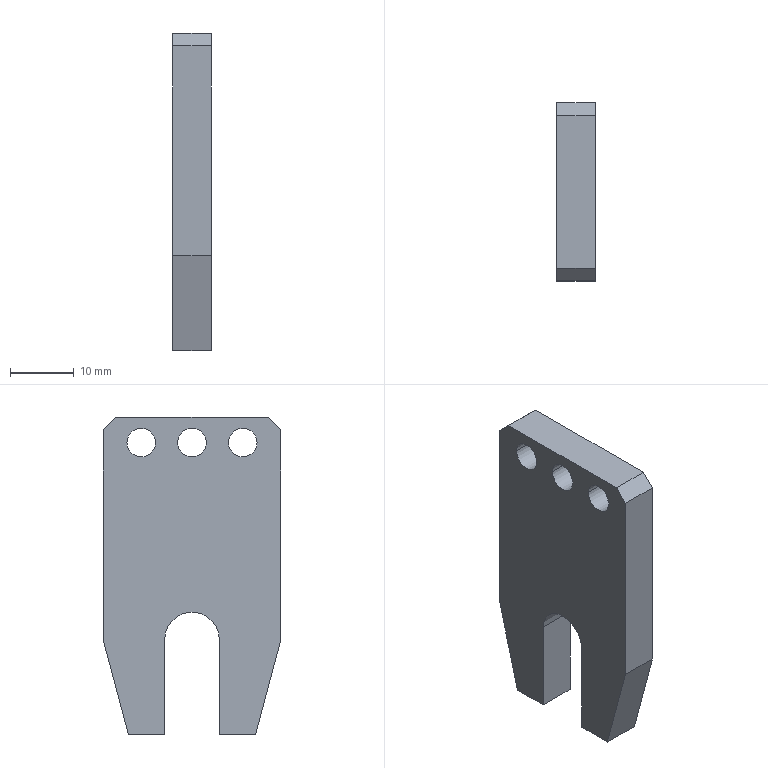Component | SolidWorks | 09HHHHHH4-1 | 1 solid | 20 faces | box 6 x 28 x 50 mm | volume 6781 mm3 | plane 13 | cylinder 7 | commonest cylinder face diameters 4.5 x6 8.6 x1
build123d program:
from build123d import *

# Parameters (mm, degrees)
SKETCH1_W           = 28
SKETCH1_H           = 50
BOSS_EXTRUDE1_DEPTH = 6
CUT_EXTRUDE1_DEPTH  = 324.627
CHAMFER1_SIZE       = 2
SKETCH3_R           = 2.25
CUT_EXTRUDE2_DEPTH  = 324.627


with BuildPart() as part:
    # Sketch1 → Boss-Extrude1 (new body)
    with BuildSketch(Plane.XY):
        with Locations((306.066, -22.5)):
            Rectangle(SKETCH1_W, SKETCH1_H)
    extrude(amount=BOSS_EXTRUDE1_DEPTH)

    # Sketch2 → Cut-Extrude1 (cut, through all)
    with BuildSketch(Plane.XY.offset(6)):
        with BuildLine():
            Line((310.366, -32.5), (310.366, -47.5))
            ThreePointArc((310.366, -47.5), (306.066, -51.8), (301.766, -47.5))
            Line((301.766, -47.5), (301.766, -32.5))
            ThreePointArc((301.766, -32.5), (306.066, -28.2), (310.366, -32.5))
        make_face()
        Polygon((296.066, -47.5), (292.066, -32.5), (292.066, -47.5), align=None)
        Polygon((320.066, -47.5), (316.066, -47.5), (320.066, -32.5), align=None)
    extrude(amount=-CUT_EXTRUDE1_DEPTH, mode=Mode.SUBTRACT)

    # Chamfer1
    chamfer1_edges = [part.edges().sort_by_distance(p)[0] for p in [
        (292.066, 2.5, 3),
        (320.066, 2.5, 3),
    ]]
    chamfer(chamfer1_edges, length=CHAMFER1_SIZE)

    # Sketch3 → Cut-Extrude2 (cut, through all)
    with BuildSketch(Plane.XY.offset(6)):
        with Locations((298.066, -1.5)):
            Circle(SKETCH3_R)
        with Locations(Location((314.066, -1.5, 0), (0, 0, 180))):
            Circle(SKETCH3_R)
        with Locations((306.066, -1.5)):
            Circle(SKETCH3_R)
    extrude(amount=-CUT_EXTRUDE2_DEPTH, mode=Mode.SUBTRACT)


solid = part.part

# Placed as in the assembly
solid = solid.moved(Location((-650.94, 19.683, 6.344), (90, -90, 0)))
STEP:
#1=CARTESIAN_POINT('',(-25.628,-11.186,0.1907));
#2=VERTEX_POINT('',#1);
#3=CARTESIAN_POINT('',(-25.628,-11.364,0.1907));
#4=VERTEX_POINT('',#3);
#5=CARTESIAN_POINT('',(-25.628,-11.275,0.1907));
#6=DIRECTION('',(-1.,0.,0.));
#7=DIRECTION('',(0.,-1.,0.));
#8=AXIS2_PLACEMENT_3D('',#5,#6,#7);
#9=CIRCLE('',#8,0.08858);
#10=EDGE_CURVE('',#2,#4,#9,.T.);
#11=ORIENTED_EDGE('',*,*,#10,.F.);
#12=CARTESIAN_POINT('',(-25.864,-11.186,0.1907));
#13=VERTEX_POINT('',#12);
#14=CARTESIAN_POINT('',(-25.628,-11.186,0.1907));
#15=DIRECTION('',(-1.,0.,0.));
#16=VECTOR('',#15,39.37);
#17=LINE('',#14,#16);
#18=EDGE_CURVE('',#2,#13,#17,.T.);
#19=ORIENTED_EDGE('',*,*,#18,.T.);
#20=CARTESIAN_POINT('',(-25.864,-11.364,0.1907));
#21=VERTEX_POINT('',#20);
#22=CARTESIAN_POINT('',(-25.864,-11.275,0.1907));
#23=DIRECTION('',(-1.,0.,0.));
#24=DIRECTION('',(0.,-1.,0.));
#25=AXIS2_PLACEMENT_3D('',#22,#23,#24);
#26=CIRCLE('',#25,0.08858);
#27=EDGE_CURVE('',#13,#21,#26,.T.);
#28=ORIENTED_EDGE('',*,*,#27,.T.);
#29=CARTESIAN_POINT('',(-25.628,-11.364,0.1907));
#30=DIRECTION('',(-1.,0.,0.));
#31=VECTOR('',#30,39.37);
#32=LINE('',#29,#31);
#33=EDGE_CURVE('',#4,#21,#32,.T.);
#34=ORIENTED_EDGE('',*,*,#33,.F.);
#35=EDGE_LOOP('',(#11,#19,#28,#34));
#36=FACE_OUTER_BOUND('',#35,.T.);
#37=CARTESIAN_POINT('',(-25.628,-11.275,0.1907));
#38=DIRECTION('',(-1.,0.,0.));
#39=DIRECTION('',(0.,-1.,0.));
#40=AXIS2_PLACEMENT_3D('',#37,#38,#39);
#41=CYLINDRICAL_SURFACE('',#40,0.08858);
#42=ADVANCED_FACE('',(#36),#41,.F.);
#43=CARTESIAN_POINT('',(-25.628,-11.501,0.1907));
#44=VERTEX_POINT('',#43);
#45=CARTESIAN_POINT('',(-25.628,-11.678,0.1907));
#46=VERTEX_POINT('',#45);
#47=CARTESIAN_POINT('',(-25.628,-11.59,0.1907));
#48=DIRECTION('',(-1.,0.,0.));
#49=DIRECTION('',(0.,1.,0.));
#50=AXIS2_PLACEMENT_3D('',#47,#48,#49);
#51=CIRCLE('',#50,0.08858);
#52=EDGE_CURVE('',#44,#46,#51,.T.);
#53=ORIENTED_EDGE('',*,*,#52,.F.);
#54=CARTESIAN_POINT('',(-25.864,-11.501,0.1907));
#55=VERTEX_POINT('',#54);
#56=CARTESIAN_POINT('',(-25.628,-11.501,0.1907));
#57=DIRECTION('',(-1.,0.,0.));
#58=VECTOR('',#57,39.37);
#59=LINE('',#56,#58);
#60=EDGE_CURVE('',#44,#55,#59,.T.);
#61=ORIENTED_EDGE('',*,*,#60,.T.);
#62=CARTESIAN_POINT('',(-25.864,-11.678,0.1907));
#63=VERTEX_POINT('',#62);
#64=CARTESIAN_POINT('',(-25.864,-11.59,0.1907));
#65=DIRECTION('',(-1.,0.,0.));
#66=DIRECTION('',(0.,1.,0.));
#67=AXIS2_PLACEMENT_3D('',#64,#65,#66);
#68=CIRCLE('',#67,0.08858);
#69=EDGE_CURVE('',#55,#63,#68,.T.);
#70=ORIENTED_EDGE('',*,*,#69,.T.);
#71=CARTESIAN_POINT('',(-25.628,-11.678,0.1907));
#72=DIRECTION('',(-1.,0.,0.));
#73=VECTOR('',#72,39.37);
#74=LINE('',#71,#73);
#75=EDGE_CURVE('',#46,#63,#74,.T.);
#76=ORIENTED_EDGE('',*,*,#75,.F.);
#77=EDGE_LOOP('',(#53,#61,#70,#76));
#78=FACE_OUTER_BOUND('',#77,.T.);
#79=CARTESIAN_POINT('',(-25.628,-11.59,0.1907));
#80=DIRECTION('',(-1.,0.,0.));
#81=DIRECTION('',(0.,-1.,0.));
#82=AXIS2_PLACEMENT_3D('',#79,#80,#81);
#83=CYLINDRICAL_SURFACE('',#82,0.08858);
#84=ADVANCED_FACE('',(#78),#83,.F.);
#85=CARTESIAN_POINT('',(-25.628,-10.871,0.1907));
#86=VERTEX_POINT('',#85);
#87=CARTESIAN_POINT('',(-25.628,-11.049,0.1907));
#88=VERTEX_POINT('',#87);
#89=CARTESIAN_POINT('',(-25.628,-10.96,0.1907));
#90=DIRECTION('',(-1.,0.,0.));
#91=DIRECTION('',(0.,-1.,0.));
#92=AXIS2_PLACEMENT_3D('',#89,#90,#91);
#93=CIRCLE('',#92,0.08858);
#94=EDGE_CURVE('',#86,#88,#93,.T.);
#95=ORIENTED_EDGE('',*,*,#94,.F.);
#96=CARTESIAN_POINT('',(-25.864,-10.871,0.1907));
#97=VERTEX_POINT('',#96);
#98=CARTESIAN_POINT('',(-25.628,-10.871,0.1907));
#99=DIRECTION('',(-1.,0.,0.));
#100=VECTOR('',#99,39.37);
#101=LINE('',#98,#100);
#102=EDGE_CURVE('',#86,#97,#101,.T.);
#103=ORIENTED_EDGE('',*,*,#102,.T.);
#104=CARTESIAN_POINT('',(-25.864,-11.049,0.1907));
#105=VERTEX_POINT('',#104);
#106=CARTESIAN_POINT('',(-25.864,-10.96,0.1907));
#107=DIRECTION('',(-1.,0.,0.));
#108=DIRECTION('',(0.,-1.,0.));
#109=AXIS2_PLACEMENT_3D('',#106,#107,#108);
#110=CIRCLE('',#109,0.08858);
#111=EDGE_CURVE('',#97,#105,#110,.T.);
#112=ORIENTED_EDGE('',*,*,#111,.T.);
#113=CARTESIAN_POINT('',(-25.628,-11.049,0.1907));
#114=DIRECTION('',(-1.,0.,0.));
#115=VECTOR('',#114,39.37);
#116=LINE('',#113,#115);
#117=EDGE_CURVE('',#88,#105,#116,.T.);
#118=ORIENTED_EDGE('',*,*,#117,.F.);
#119=EDGE_LOOP('',(#95,#103,#112,#118));
#120=FACE_OUTER_BOUND('',#119,.T.);
#121=CARTESIAN_POINT('',(-25.628,-10.96,0.1907));
#122=DIRECTION('',(-1.,0.,0.));
#123=DIRECTION('',(0.,-1.,0.));
#124=AXIS2_PLACEMENT_3D('',#121,#122,#123);
#125=CYLINDRICAL_SURFACE('',#124,0.08858);
#126=ADVANCED_FACE('',(#120),#125,.F.);
#127=CARTESIAN_POINT('',(-25.628,-11.444,-1.62));
#128=VERTEX_POINT('',#127);
#129=CARTESIAN_POINT('',(-25.628,-11.669,-1.62));
#130=VERTEX_POINT('',#129);
#131=CARTESIAN_POINT('',(-25.628,-10.724,-1.62));
#132=DIRECTION('',(0.,-1.,0.));
#133=VECTOR('',#132,39.37);
#134=LINE('',#131,#133);
#135=EDGE_CURVE('',#128,#130,#134,.T.);
#136=ORIENTED_EDGE('',*,*,#135,.T.);
#137=CARTESIAN_POINT('',(-25.864,-11.669,-1.62));
#138=VERTEX_POINT('',#137);
#139=CARTESIAN_POINT('',(-25.628,-11.669,-1.62));
#140=DIRECTION('',(-1.,0.,0.));
#141=VECTOR('',#140,39.37);
#142=LINE('',#139,#141);
#143=EDGE_CURVE('',#130,#138,#142,.T.);
#144=ORIENTED_EDGE('',*,*,#143,.T.);
#145=CARTESIAN_POINT('',(-25.864,-11.444,-1.62));
#146=VERTEX_POINT('',#145);
#147=CARTESIAN_POINT('',(-25.864,-10.724,-1.62));
#148=DIRECTION('',(0.,-1.,0.));
#149=VECTOR('',#148,39.37);
#150=LINE('',#147,#149);
#151=EDGE_CURVE('',#146,#138,#150,.T.);
#152=ORIENTED_EDGE('',*,*,#151,.F.);
#153=CARTESIAN_POINT('',(-25.628,-11.444,-1.62));
#154=DIRECTION('',(-1.,0.,0.));
#155=VECTOR('',#154,39.37);
#156=LINE('',#153,#155);
#157=EDGE_CURVE('',#128,#146,#156,.T.);
#158=ORIENTED_EDGE('',*,*,#157,.F.);
#159=EDGE_LOOP('',(#136,#144,#152,#158));
#160=FACE_OUTER_BOUND('',#159,.T.);
#161=CARTESIAN_POINT('',(-25.864,-10.724,-1.62));
#162=DIRECTION('',(0.,0.,1.));
#163=DIRECTION('',(-1.,0.,0.));
#164=AXIS2_PLACEMENT_3D('',#161,#162,#163);
#165=PLANE('',#164);
#166=ADVANCED_FACE('',(#160),#165,.F.);
#167=CARTESIAN_POINT('',(-25.864,-10.724,0.2694));
#168=VERTEX_POINT('',#167);
#169=CARTESIAN_POINT('',(-25.864,-10.724,-1.03));
#170=VERTEX_POINT('',#169);
#171=CARTESIAN_POINT('',(-25.864,-10.724,0.3482));
#172=DIRECTION('',(0.,0.,-1.));
#173=VECTOR('',#172,39.37);
#174=LINE('',#171,#173);
#175=EDGE_CURVE('',#168,#170,#174,.T.);
#176=ORIENTED_EDGE('',*,*,#175,.F.);
#177=CARTESIAN_POINT('',(-25.628,-10.724,0.2694));
#178=VERTEX_POINT('',#177);
#179=CARTESIAN_POINT('',(-25.864,-10.724,0.2694));
#180=DIRECTION('',(1.,0.,0.));
#181=VECTOR('',#180,39.37);
#182=LINE('',#179,#181);
#183=EDGE_CURVE('',#168,#178,#182,.T.);
#184=ORIENTED_EDGE('',*,*,#183,.T.);
#185=CARTESIAN_POINT('',(-25.628,-10.724,-1.03));
#186=VERTEX_POINT('',#185);
#187=CARTESIAN_POINT('',(-25.628,-10.724,0.3482));
#188=DIRECTION('',(0.,0.,-1.));
#189=VECTOR('',#188,39.37);
#190=LINE('',#187,#189);
#191=EDGE_CURVE('',#178,#186,#190,.T.);
#192=ORIENTED_EDGE('',*,*,#191,.T.);
#193=CARTESIAN_POINT('',(-25.628,-10.724,-1.03));
#194=DIRECTION('',(-1.,0.,0.));
#195=VECTOR('',#194,39.37);
#196=LINE('',#193,#195);
#197=EDGE_CURVE('',#186,#170,#196,.T.);
#198=ORIENTED_EDGE('',*,*,#197,.T.);
#199=EDGE_LOOP('',(#176,#184,#192,#198));
#200=FACE_OUTER_BOUND('',#199,.T.);
#201=CARTESIAN_POINT('',(-25.864,-10.724,0.3482));
#202=DIRECTION('',(0.,-1.,0.));
#203=DIRECTION('',(1.,0.,0.));
#204=AXIS2_PLACEMENT_3D('',#201,#202,#203);
#205=PLANE('',#204);
#206=ADVANCED_FACE('',(#200),#205,.F.);
#207=CARTESIAN_POINT('',(-25.864,-10.881,-1.62));
#208=VERTEX_POINT('',#207);
#209=CARTESIAN_POINT('',(-25.864,-11.106,-1.62));
#210=VERTEX_POINT('',#209);
#211=CARTESIAN_POINT('',(-25.864,-10.724,-1.62));
#212=DIRECTION('',(0.,-1.,0.));
#213=VECTOR('',#212,39.37);
#214=LINE('',#211,#213);
#215=EDGE_CURVE('',#208,#210,#214,.T.);
#216=ORIENTED_EDGE('',*,*,#215,.F.);
#217=CARTESIAN_POINT('',(-25.628,-10.881,-1.62));
#218=VERTEX_POINT('',#217);
#219=CARTESIAN_POINT('',(-25.628,-10.881,-1.62));
#220=DIRECTION('',(-1.,0.,0.));
#221=VECTOR('',#220,39.37);
#222=LINE('',#219,#221);
#223=EDGE_CURVE('',#218,#208,#222,.T.);
#224=ORIENTED_EDGE('',*,*,#223,.F.);
#225=CARTESIAN_POINT('',(-25.628,-11.106,-1.62));
#226=VERTEX_POINT('',#225);
#227=CARTESIAN_POINT('',(-25.628,-10.724,-1.62));
#228=DIRECTION('',(0.,-1.,0.));
#229=VECTOR('',#228,39.37);
#230=LINE('',#227,#229);
#231=EDGE_CURVE('',#218,#226,#230,.T.);
#232=ORIENTED_EDGE('',*,*,#231,.T.);
#233=CARTESIAN_POINT('',(-25.628,-11.106,-1.62));
#234=DIRECTION('',(-1.,0.,0.));
#235=VECTOR('',#234,39.37);
#236=LINE('',#233,#235);
#237=EDGE_CURVE('',#226,#210,#236,.T.);
#238=ORIENTED_EDGE('',*,*,#237,.T.);
#239=EDGE_LOOP('',(#216,#224,#232,#238));
#240=FACE_OUTER_BOUND('',#239,.T.);
#241=CARTESIAN_POINT('',(-25.864,-10.724,-1.62));
#242=DIRECTION('',(0.,0.,1.));
#243=DIRECTION('',(-1.,0.,0.));
#244=AXIS2_PLACEMENT_3D('',#241,#242,#243);
#245=PLANE('',#244);
#246=ADVANCED_FACE('',(#240),#245,.F.);
#247=CARTESIAN_POINT('',(-25.628,-11.826,-1.03));
#248=VERTEX_POINT('',#247);
#249=CARTESIAN_POINT('',(-25.628,-11.826,0.2694));
#250=VERTEX_POINT('',#249);
#251=CARTESIAN_POINT('',(-25.628,-11.826,0.3482));
#252=DIRECTION('',(0.,0.,1.));
#253=VECTOR('',#252,39.37);
#254=LINE('',#251,#253);
#255=EDGE_CURVE('',#248,#250,#254,.T.);
#256=ORIENTED_EDGE('',*,*,#255,.T.);
#257=CARTESIAN_POINT('',(-25.864,-11.826,0.2694));
#258=VERTEX_POINT('',#257);
#259=CARTESIAN_POINT('',(-25.864,-11.826,0.2694));
#260=DIRECTION('',(-1.,0.,0.));
#261=VECTOR('',#260,39.37);
#262=LINE('',#259,#261);
#263=EDGE_CURVE('',#250,#258,#262,.T.);
#264=ORIENTED_EDGE('',*,*,#263,.T.);
#265=CARTESIAN_POINT('',(-25.864,-11.826,-1.03));
#266=VERTEX_POINT('',#265);
#267=CARTESIAN_POINT('',(-25.864,-11.826,0.3482));
#268=DIRECTION('',(0.,0.,1.));
#269=VECTOR('',#268,39.37);
#270=LINE('',#267,#269);
#271=EDGE_CURVE('',#266,#258,#270,.T.);
#272=ORIENTED_EDGE('',*,*,#271,.F.);
#273=CARTESIAN_POINT('',(-25.628,-11.826,-1.03));
#274=DIRECTION('',(-1.,0.,0.));
#275=VECTOR('',#274,39.37);
#276=LINE('',#273,#275);
#277=EDGE_CURVE('',#248,#266,#276,.T.);
#278=ORIENTED_EDGE('',*,*,#277,.F.);
#279=EDGE_LOOP('',(#256,#264,#272,#278));
#280=FACE_OUTER_BOUND('',#279,.T.);
#281=CARTESIAN_POINT('',(-25.864,-11.826,0.3482));
#282=DIRECTION('',(0.,1.,0.));
#283=DIRECTION('',(-1.,0.,0.));
#284=AXIS2_PLACEMENT_3D('',#281,#282,#283);
#285=PLANE('',#284);
#286=ADVANCED_FACE('',(#280),#285,.F.);
#287=CARTESIAN_POINT('',(-25.864,-11.747,0.3482));
#288=VERTEX_POINT('',#287);
#289=CARTESIAN_POINT('',(-25.864,-10.802,0.3482));
#290=VERTEX_POINT('',#289);
#291=CARTESIAN_POINT('',(-25.864,-10.724,0.3482));
#292=DIRECTION('',(0.,1.,0.));
#293=VECTOR('',#292,39.37);
#294=LINE('',#291,#293);
#295=EDGE_CURVE('',#288,#290,#294,.T.);
#296=ORIENTED_EDGE('',*,*,#295,.F.);
#297=CARTESIAN_POINT('',(-25.628,-11.747,0.3482));
#298=VERTEX_POINT('',#297);
#299=CARTESIAN_POINT('',(-25.864,-11.747,0.3482));
#300=DIRECTION('',(1.,0.,0.));
#301=VECTOR('',#300,39.37);
#302=LINE('',#299,#301);
#303=EDGE_CURVE('',#288,#298,#302,.T.);
#304=ORIENTED_EDGE('',*,*,#303,.T.);
#305=CARTESIAN_POINT('',(-25.628,-10.802,0.3482));
#306=VERTEX_POINT('',#305);
#307=CARTESIAN_POINT('',(-25.628,-10.724,0.3482));
#308=DIRECTION('',(0.,1.,0.));
#309=VECTOR('',#308,39.37);
#310=LINE('',#307,#309);
#311=EDGE_CURVE('',#298,#306,#310,.T.);
#312=ORIENTED_EDGE('',*,*,#311,.T.);
#313=CARTESIAN_POINT('',(-25.864,-10.802,0.3482));
#314=DIRECTION('',(-1.,0.,0.));
#315=VECTOR('',#314,39.37);
#316=LINE('',#313,#315);
#317=EDGE_CURVE('',#306,#290,#316,.T.);
#318=ORIENTED_EDGE('',*,*,#317,.T.);
#319=EDGE_LOOP('',(#296,#304,#312,#318));
#320=FACE_OUTER_BOUND('',#319,.T.);
#321=CARTESIAN_POINT('',(-25.864,-10.724,0.3482));
#322=DIRECTION('',(0.,0.,-1.));
#323=DIRECTION('',(1.,0.,0.));
#324=AXIS2_PLACEMENT_3D('',#321,#322,#323);
#325=PLANE('',#324);
#326=ADVANCED_FACE('',(#320),#325,.F.);
#327=CARTESIAN_POINT('',(-25.864,-11.275,0.1907));
#328=DIRECTION('',(-1.,0.,0.));
#329=DIRECTION('',(0.,-1.,0.));
#330=AXIS2_PLACEMENT_3D('',#327,#328,#329);
#331=CIRCLE('',#330,0.08858);
#332=EDGE_CURVE('',#21,#13,#331,.T.);
#333=ORIENTED_EDGE('',*,*,#332,.F.);
#334=ORIENTED_EDGE('',*,*,#27,.F.);
#335=EDGE_LOOP('',(#333,#334));
#336=FACE_BOUND('',#335,.T.);
#337=CARTESIAN_POINT('',(-25.864,-11.59,0.1907));
#338=DIRECTION('',(-1.,0.,0.));
#339=DIRECTION('',(0.,1.,0.));
#340=AXIS2_PLACEMENT_3D('',#337,#338,#339);
#341=CIRCLE('',#340,0.08858);
#342=EDGE_CURVE('',#63,#55,#341,.T.);
#343=ORIENTED_EDGE('',*,*,#342,.F.);
#344=ORIENTED_EDGE('',*,*,#69,.F.);
#345=EDGE_LOOP('',(#343,#344));
#346=FACE_BOUND('',#345,.T.);
#347=CARTESIAN_POINT('',(-25.864,-10.96,0.1907));
#348=DIRECTION('',(-1.,0.,0.));
#349=DIRECTION('',(0.,-1.,0.));
#350=AXIS2_PLACEMENT_3D('',#347,#348,#349);
#351=CIRCLE('',#350,0.08858);
#352=EDGE_CURVE('',#105,#97,#351,.T.);
#353=ORIENTED_EDGE('',*,*,#352,.F.);
#354=ORIENTED_EDGE('',*,*,#111,.F.);
#355=EDGE_LOOP('',(#353,#354));
#356=FACE_BOUND('',#355,.T.);
#357=ORIENTED_EDGE('',*,*,#271,.T.);
#358=CARTESIAN_POINT('',(-25.864,-5.535,6.56));
#359=DIRECTION('',(0.,0.7071,0.7071));
#360=VECTOR('',#359,39.37);
#361=LINE('',#358,#360);
#362=EDGE_CURVE('',#258,#288,#361,.T.);
#363=ORIENTED_EDGE('',*,*,#362,.T.);
#364=ORIENTED_EDGE('',*,*,#295,.T.);
#365=CARTESIAN_POINT('',(-25.864,-4.965,-5.49));
#366=DIRECTION('',(0.,0.7071,-0.7071));
#367=VECTOR('',#366,39.37);
#368=LINE('',#365,#367);
#369=EDGE_CURVE('',#290,#168,#368,.T.);
#370=ORIENTED_EDGE('',*,*,#369,.T.);
#371=ORIENTED_EDGE('',*,*,#175,.T.);
#372=CARTESIAN_POINT('',(-25.864,-10.881,-1.62));
#373=DIRECTION('',(0.,0.2577,0.9662));
#374=VECTOR('',#373,39.37);
#375=LINE('',#372,#374);
#376=EDGE_CURVE('',#208,#170,#375,.T.);
#377=ORIENTED_EDGE('',*,*,#376,.F.);
#378=ORIENTED_EDGE('',*,*,#215,.T.);
#379=CARTESIAN_POINT('',(-25.864,-11.106,-1.03));
#380=VERTEX_POINT('',#379);
#381=CARTESIAN_POINT('',(-25.864,-11.106,-1.03));
#382=DIRECTION('',(0.,0.,-1.));
#383=VECTOR('',#382,39.37);
#384=LINE('',#381,#383);
#385=EDGE_CURVE('',#380,#210,#384,.T.);
#386=ORIENTED_EDGE('',*,*,#385,.F.);
#387=CARTESIAN_POINT('',(-25.864,-11.444,-1.03));
#388=VERTEX_POINT('',#387);
#389=CARTESIAN_POINT('',(-25.864,-11.275,-1.03));
#390=DIRECTION('',(-1.,0.,0.));
#391=DIRECTION('',(0.,-1.,0.));
#392=AXIS2_PLACEMENT_3D('',#389,#390,#391);
#393=CIRCLE('',#392,0.1693);
#394=EDGE_CURVE('',#388,#380,#393,.T.);
#395=ORIENTED_EDGE('',*,*,#394,.F.);
#396=CARTESIAN_POINT('',(-25.864,-11.444,-1.03));
#397=DIRECTION('',(0.,0.,1.));
#398=VECTOR('',#397,39.37);
#399=LINE('',#396,#398);
#400=EDGE_CURVE('',#146,#388,#399,.T.);
#401=ORIENTED_EDGE('',*,*,#400,.F.);
#402=ORIENTED_EDGE('',*,*,#151,.T.);
#403=CARTESIAN_POINT('',(-25.864,-11.669,-1.62));
#404=DIRECTION('',(0.,0.2577,-0.9662));
#405=VECTOR('',#404,39.37);
#406=LINE('',#403,#405);
#407=EDGE_CURVE('',#266,#138,#406,.T.);
#408=ORIENTED_EDGE('',*,*,#407,.F.);
#409=EDGE_LOOP('',(#357,#363,#364,#370,#371,#377,#378,#386,#395,#401,#402,#408));
#410=FACE_OUTER_BOUND('',#409,.T.);
#411=CARTESIAN_POINT('',(-25.864,0.7749,0.2498));
#412=DIRECTION('',(-1.,0.,0.));
#413=DIRECTION('',(0.,-1.,0.));
#414=AXIS2_PLACEMENT_3D('',#411,#412,#413);
#415=PLANE('',#414);
#416=ADVANCED_FACE('',(#336,#346,#356,#410),#415,.T.);
#417=CARTESIAN_POINT('',(-25.628,-11.275,0.1907));
#418=DIRECTION('',(-1.,0.,0.));
#419=DIRECTION('',(0.,-1.,0.));
#420=AXIS2_PLACEMENT_3D('',#417,#418,#419);
#421=CIRCLE('',#420,0.08858);
#422=EDGE_CURVE('',#4,#2,#421,.T.);
#423=ORIENTED_EDGE('',*,*,#422,.T.);
#424=ORIENTED_EDGE('',*,*,#10,.T.);
#425=EDGE_LOOP('',(#423,#424));
#426=FACE_BOUND('',#425,.T.);
#427=CARTESIAN_POINT('',(-25.628,-11.59,0.1907));
#428=DIRECTION('',(-1.,0.,0.));
#429=DIRECTION('',(0.,1.,0.));
#430=AXIS2_PLACEMENT_3D('',#427,#428,#429);
#431=CIRCLE('',#430,0.08858);
#432=EDGE_CURVE('',#46,#44,#431,.T.);
#433=ORIENTED_EDGE('',*,*,#432,.T.);
#434=ORIENTED_EDGE('',*,*,#52,.T.);
#435=EDGE_LOOP('',(#433,#434));
#436=FACE_BOUND('',#435,.T.);
#437=CARTESIAN_POINT('',(-25.628,-10.96,0.1907));
#438=DIRECTION('',(-1.,0.,0.));
#439=DIRECTION('',(0.,-1.,0.));
#440=AXIS2_PLACEMENT_3D('',#437,#438,#439);
#441=CIRCLE('',#440,0.08858);
#442=EDGE_CURVE('',#88,#86,#441,.T.);
#443=ORIENTED_EDGE('',*,*,#442,.T.);
#444=ORIENTED_EDGE('',*,*,#94,.T.);
#445=EDGE_LOOP('',(#443,#444));
#446=FACE_BOUND('',#445,.T.);
#447=ORIENTED_EDGE('',*,*,#311,.F.);
#448=CARTESIAN_POINT('',(-25.628,-11.747,0.3482));
#449=DIRECTION('',(0.,-0.7071,-0.7071));
#450=VECTOR('',#449,39.37);
#451=LINE('',#448,#450);
#452=EDGE_CURVE('',#298,#250,#451,.T.);
#453=ORIENTED_EDGE('',*,*,#452,.T.);
#454=ORIENTED_EDGE('',*,*,#255,.F.);
#455=CARTESIAN_POINT('',(-25.628,-11.669,-1.62));
#456=DIRECTION('',(0.,0.2577,-0.9662));
#457=VECTOR('',#456,39.37);
#458=LINE('',#455,#457);
#459=EDGE_CURVE('',#248,#130,#458,.T.);
#460=ORIENTED_EDGE('',*,*,#459,.T.);
#461=ORIENTED_EDGE('',*,*,#135,.F.);
#462=CARTESIAN_POINT('',(-25.628,-11.444,-1.03));
#463=VERTEX_POINT('',#462);
#464=CARTESIAN_POINT('',(-25.628,-11.444,-1.03));
#465=DIRECTION('',(0.,0.,1.));
#466=VECTOR('',#465,39.37);
#467=LINE('',#464,#466);
#468=EDGE_CURVE('',#128,#463,#467,.T.);
#469=ORIENTED_EDGE('',*,*,#468,.T.);
#470=CARTESIAN_POINT('',(-25.628,-11.106,-1.03));
#471=VERTEX_POINT('',#470);
#472=CARTESIAN_POINT('',(-25.628,-11.275,-1.03));
#473=DIRECTION('',(-1.,0.,0.));
#474=DIRECTION('',(0.,-1.,0.));
#475=AXIS2_PLACEMENT_3D('',#472,#473,#474);
#476=CIRCLE('',#475,0.1693);
#477=EDGE_CURVE('',#463,#471,#476,.T.);
#478=ORIENTED_EDGE('',*,*,#477,.T.);
#479=CARTESIAN_POINT('',(-25.628,-11.106,-1.03));
#480=DIRECTION('',(0.,0.,-1.));
#481=VECTOR('',#480,39.37);
#482=LINE('',#479,#481);
#483=EDGE_CURVE('',#471,#226,#482,.T.);
#484=ORIENTED_EDGE('',*,*,#483,.T.);
#485=ORIENTED_EDGE('',*,*,#231,.F.);
#486=CARTESIAN_POINT('',(-25.628,-10.881,-1.62));
#487=DIRECTION('',(0.,0.2577,0.9662));
#488=VECTOR('',#487,39.37);
#489=LINE('',#486,#488);
#490=EDGE_CURVE('',#218,#186,#489,.T.);
#491=ORIENTED_EDGE('',*,*,#490,.T.);
#492=ORIENTED_EDGE('',*,*,#191,.F.);
#493=CARTESIAN_POINT('',(-25.628,-10.724,0.2694));
#494=DIRECTION('',(0.,-0.7071,0.7071));
#495=VECTOR('',#494,39.37);
#496=LINE('',#493,#495);
#497=EDGE_CURVE('',#178,#306,#496,.T.);
#498=ORIENTED_EDGE('',*,*,#497,.T.);
#499=EDGE_LOOP('',(#447,#453,#454,#460,#461,#469,#478,#484,#485,#491,#492,#498));
#500=FACE_OUTER_BOUND('',#499,.T.);
#501=CARTESIAN_POINT('',(-25.628,0.7749,0.2498));
#502=DIRECTION('',(-1.,0.,0.));
#503=DIRECTION('',(0.,-1.,0.));
#504=AXIS2_PLACEMENT_3D('',#501,#502,#503);
#505=PLANE('',#504);
#506=ADVANCED_FACE('',(#426,#436,#446,#500),#505,.F.);
#507=ORIENTED_EDGE('',*,*,#394,.T.);
#508=CARTESIAN_POINT('',(-25.628,-11.106,-1.03));
#509=DIRECTION('',(-1.,0.,0.));
#510=VECTOR('',#509,39.37);
#511=LINE('',#508,#510);
#512=EDGE_CURVE('',#471,#380,#511,.T.);
#513=ORIENTED_EDGE('',*,*,#512,.F.);
#514=ORIENTED_EDGE('',*,*,#477,.F.);
#515=CARTESIAN_POINT('',(-25.628,-11.444,-1.03));
#516=DIRECTION('',(-1.,0.,0.));
#517=VECTOR('',#516,39.37);
#518=LINE('',#515,#517);
#519=EDGE_CURVE('',#463,#388,#518,.T.);
#520=ORIENTED_EDGE('',*,*,#519,.T.);
#521=EDGE_LOOP('',(#507,#513,#514,#520));
#522=FACE_OUTER_BOUND('',#521,.T.);
#523=CARTESIAN_POINT('',(-25.628,-11.275,-1.03));
#524=DIRECTION('',(-1.,0.,0.));
#525=DIRECTION('',(0.,-1.,0.));
#526=AXIS2_PLACEMENT_3D('',#523,#524,#525);
#527=CYLINDRICAL_SURFACE('',#526,0.1693);
#528=ADVANCED_FACE('',(#522),#527,.F.);
#529=ORIENTED_EDGE('',*,*,#400,.T.);
#530=ORIENTED_EDGE('',*,*,#519,.F.);
#531=ORIENTED_EDGE('',*,*,#468,.F.);
#532=ORIENTED_EDGE('',*,*,#157,.T.);
#533=EDGE_LOOP('',(#529,#530,#531,#532));
#534=FACE_OUTER_BOUND('',#533,.T.);
#535=CARTESIAN_POINT('',(-25.628,-11.444,-1.03));
#536=DIRECTION('',(0.,-1.,0.));
#537=DIRECTION('',(0.,0.,1.));
#538=AXIS2_PLACEMENT_3D('',#535,#536,#537);
#539=PLANE('',#538);
#540=ADVANCED_FACE('',(#534),#539,.F.);
#541=ORIENTED_EDGE('',*,*,#385,.T.);
#542=ORIENTED_EDGE('',*,*,#237,.F.);
#543=ORIENTED_EDGE('',*,*,#483,.F.);
#544=ORIENTED_EDGE('',*,*,#512,.T.);
#545=EDGE_LOOP('',(#541,#542,#543,#544));
#546=FACE_OUTER_BOUND('',#545,.T.);
#547=CARTESIAN_POINT('',(-25.628,-11.106,-1.03));
#548=DIRECTION('',(0.,1.,0.));
#549=DIRECTION('',(0.,0.,-1.));
#550=AXIS2_PLACEMENT_3D('',#547,#548,#549);
#551=PLANE('',#550);
#552=ADVANCED_FACE('',(#546),#551,.F.);
#553=ORIENTED_EDGE('',*,*,#376,.T.);
#554=ORIENTED_EDGE('',*,*,#197,.F.);
#555=ORIENTED_EDGE('',*,*,#490,.F.);
#556=ORIENTED_EDGE('',*,*,#223,.T.);
#557=EDGE_LOOP('',(#553,#554,#555,#556));
#558=FACE_OUTER_BOUND('',#557,.T.);
#559=CARTESIAN_POINT('',(-25.628,-10.881,-1.62));
#560=DIRECTION('',(0.,-0.9662,0.2577));
#561=DIRECTION('',(0.,0.2577,0.9662));
#562=AXIS2_PLACEMENT_3D('',#559,#560,#561);
#563=PLANE('',#562);
#564=ADVANCED_FACE('',(#558),#563,.F.);
#565=ORIENTED_EDGE('',*,*,#407,.T.);
#566=ORIENTED_EDGE('',*,*,#143,.F.);
#567=ORIENTED_EDGE('',*,*,#459,.F.);
#568=ORIENTED_EDGE('',*,*,#277,.T.);
#569=EDGE_LOOP('',(#565,#566,#567,#568));
#570=FACE_OUTER_BOUND('',#569,.T.);
#571=CARTESIAN_POINT('',(-25.628,-11.669,-1.62));
#572=DIRECTION('',(0.,0.9662,0.2577));
#573=DIRECTION('',(0.,0.2577,-0.9662));
#574=AXIS2_PLACEMENT_3D('',#571,#572,#573);
#575=PLANE('',#574);
#576=ADVANCED_FACE('',(#570),#575,.F.);
#577=ORIENTED_EDGE('',*,*,#362,.F.);
#578=ORIENTED_EDGE('',*,*,#263,.F.);
#579=ORIENTED_EDGE('',*,*,#452,.F.);
#580=ORIENTED_EDGE('',*,*,#303,.F.);
#581=EDGE_LOOP('',(#577,#578,#579,#580));
#582=FACE_OUTER_BOUND('',#581,.T.);
#583=CARTESIAN_POINT('',(-25.864,-11.747,0.3482));
#584=DIRECTION('',(0.,0.7071,-0.7071));
#585=DIRECTION('',(1.,0.,0.));
#586=AXIS2_PLACEMENT_3D('',#583,#584,#585);
#587=PLANE('',#586);
#588=ADVANCED_FACE('',(#582),#587,.F.);
#589=ORIENTED_EDGE('',*,*,#369,.F.);
#590=ORIENTED_EDGE('',*,*,#317,.F.);
#591=ORIENTED_EDGE('',*,*,#497,.F.);
#592=ORIENTED_EDGE('',*,*,#183,.F.);
#593=EDGE_LOOP('',(#589,#590,#591,#592));
#594=FACE_OUTER_BOUND('',#593,.T.);
#595=CARTESIAN_POINT('',(-25.864,-10.724,0.2694));
#596=DIRECTION('',(0.,-0.7071,-0.7071));
#597=DIRECTION('',(1.,0.,0.));
#598=AXIS2_PLACEMENT_3D('',#595,#596,#597);
#599=PLANE('',#598);
#600=ADVANCED_FACE('',(#594),#599,.F.);
#601=ORIENTED_EDGE('',*,*,#102,.F.);
#602=ORIENTED_EDGE('',*,*,#442,.F.);
#603=ORIENTED_EDGE('',*,*,#117,.T.);
#604=ORIENTED_EDGE('',*,*,#352,.T.);
#605=EDGE_LOOP('',(#601,#602,#603,#604));
#606=FACE_OUTER_BOUND('',#605,.T.);
#607=CARTESIAN_POINT('',(-25.628,-10.96,0.1907));
#608=DIRECTION('',(-1.,0.,0.));
#609=DIRECTION('',(0.,-1.,0.));
#610=AXIS2_PLACEMENT_3D('',#607,#608,#609);
#611=CYLINDRICAL_SURFACE('',#610,0.08858);
#612=ADVANCED_FACE('',(#606),#611,.F.);
#613=ORIENTED_EDGE('',*,*,#60,.F.);
#614=ORIENTED_EDGE('',*,*,#432,.F.);
#615=ORIENTED_EDGE('',*,*,#75,.T.);
#616=ORIENTED_EDGE('',*,*,#342,.T.);
#617=EDGE_LOOP('',(#613,#614,#615,#616));
#618=FACE_OUTER_BOUND('',#617,.T.);
#619=CARTESIAN_POINT('',(-25.628,-11.59,0.1907));
#620=DIRECTION('',(-1.,0.,0.));
#621=DIRECTION('',(0.,-1.,0.));
#622=AXIS2_PLACEMENT_3D('',#619,#620,#621);
#623=CYLINDRICAL_SURFACE('',#622,0.08858);
#624=ADVANCED_FACE('',(#618),#623,.F.);
#625=ORIENTED_EDGE('',*,*,#18,.F.);
#626=ORIENTED_EDGE('',*,*,#422,.F.);
#627=ORIENTED_EDGE('',*,*,#33,.T.);
#628=ORIENTED_EDGE('',*,*,#332,.T.);
#629=EDGE_LOOP('',(#625,#626,#627,#628));
#630=FACE_OUTER_BOUND('',#629,.T.);
#631=CARTESIAN_POINT('',(-25.628,-11.275,0.1907));
#632=DIRECTION('',(-1.,0.,0.));
#633=DIRECTION('',(0.,-1.,0.));
#634=AXIS2_PLACEMENT_3D('',#631,#632,#633);
#635=CYLINDRICAL_SURFACE('',#634,0.08858);
#636=ADVANCED_FACE('',(#630),#635,.F.);
#637=CLOSED_SHELL('',(#42,#84,#126,#166,#206,#246,#286,#326,#416,#506,#528,#540,#552,#564,#576,#588,#600,#612,#624,#636));
#638=MANIFOLD_SOLID_BREP('',#637);
#639=CARTESIAN_POINT('',(0.,0.,0.));
#640=DIRECTION('',(0.,0.,1.));
#641=DIRECTION('',(1.,0.,0.));
#642=AXIS2_PLACEMENT_3D('',#639,#640,#641);
#643=(LENGTH_UNIT()NAMED_UNIT(*)SI_UNIT($,.METRE.));
#644=LENGTH_MEASURE_WITH_UNIT(LENGTH_MEASURE(0.0254),#643);
#645=DIMENSIONAL_EXPONENTS(1.,0.,0.,0.,0.,0.,0.);
#646=(CONVERSION_BASED_UNIT('',#644)LENGTH_UNIT()NAMED_UNIT(#645));
#647=UNCERTAINTY_MEASURE_WITH_UNIT(LENGTH_MEASURE(0.00001),#646,'','');
#648=(NAMED_UNIT(*)PLANE_ANGLE_UNIT()SI_UNIT($,.RADIAN.));
#649=(NAMED_UNIT(*)SI_UNIT($,.STERADIAN.)SOLID_ANGLE_UNIT());
#650=(GEOMETRIC_REPRESENTATION_CONTEXT(3)GLOBAL_UNCERTAINTY_ASSIGNED_CONTEXT((#647))GLOBAL_UNIT_ASSIGNED_CONTEXT((#646,#648,#649))REPRESENTATION_CONTEXT('',''));
#651=ADVANCED_BREP_SHAPE_REPRESENTATION('',(#638,#642),#650);
#652=COLOUR_RGB('',0.7922,0.8196,0.9333);
#653=FILL_AREA_STYLE_COLOUR('',#652);
#654=FILL_AREA_STYLE('',(#653));
#655=SURFACE_STYLE_FILL_AREA(#654);
#656=SURFACE_SIDE_STYLE('',(#655));
#657=SURFACE_STYLE_USAGE(.BOTH.,#656);
#658=PRESENTATION_STYLE_ASSIGNMENT((#657));
#659=STYLED_ITEM('',(#658),#638);
#660=(LENGTH_UNIT()NAMED_UNIT(*)SI_UNIT($,.METRE.));
#661=LENGTH_MEASURE_WITH_UNIT(LENGTH_MEASURE(0.0254),#660);
#662=DIMENSIONAL_EXPONENTS(1.,0.,0.,0.,0.,0.,0.);
#663=(CONVERSION_BASED_UNIT('',#661)LENGTH_UNIT()NAMED_UNIT(#662));
#664=UNCERTAINTY_MEASURE_WITH_UNIT(LENGTH_MEASURE(0.00001),#663,'','');
#665=(NAMED_UNIT(*)PLANE_ANGLE_UNIT()SI_UNIT($,.RADIAN.));
#666=(NAMED_UNIT(*)SI_UNIT($,.STERADIAN.)SOLID_ANGLE_UNIT());
#667=(GEOMETRIC_REPRESENTATION_CONTEXT(3)GLOBAL_UNCERTAINTY_ASSIGNED_CONTEXT((#664))GLOBAL_UNIT_ASSIGNED_CONTEXT((#663,#665,#666))REPRESENTATION_CONTEXT('',''));
#668=MECHANICAL_DESIGN_GEOMETRIC_PRESENTATION_REPRESENTATION('',(#659),#667);
#669=PRESENTATION_LAYER_ASSIGNMENT('','',(#659));